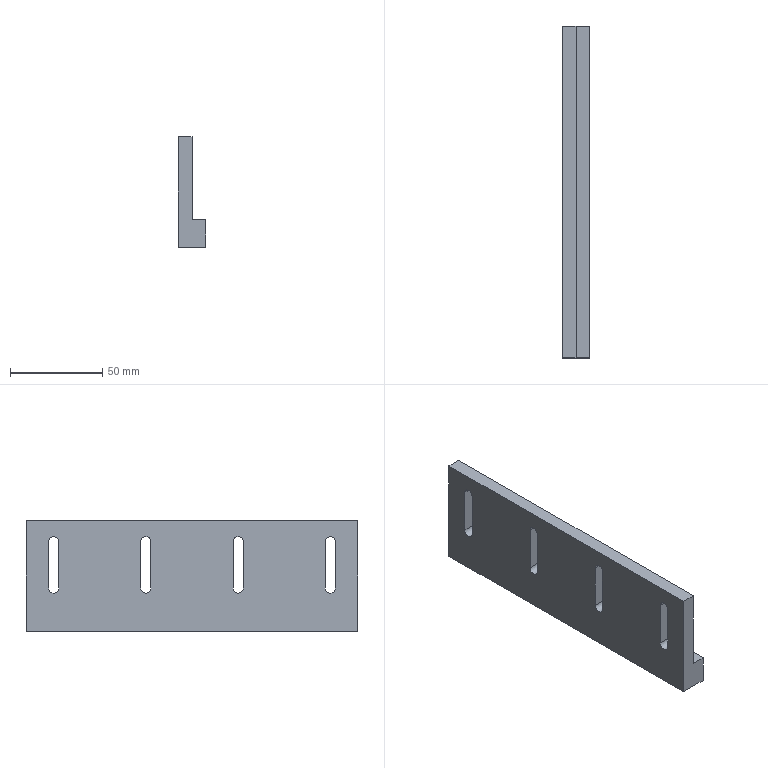Component | SolidWorks | P-SLJ-001-004-1 | 1 solid | 44 faces | box 15 x 180 x 60 mm | volume 95613 mm3 | cylinder 20 | plane 16 | cone 8 | commonest cylinder face diameters 5.5 x12 4.2 x8 | material 45#